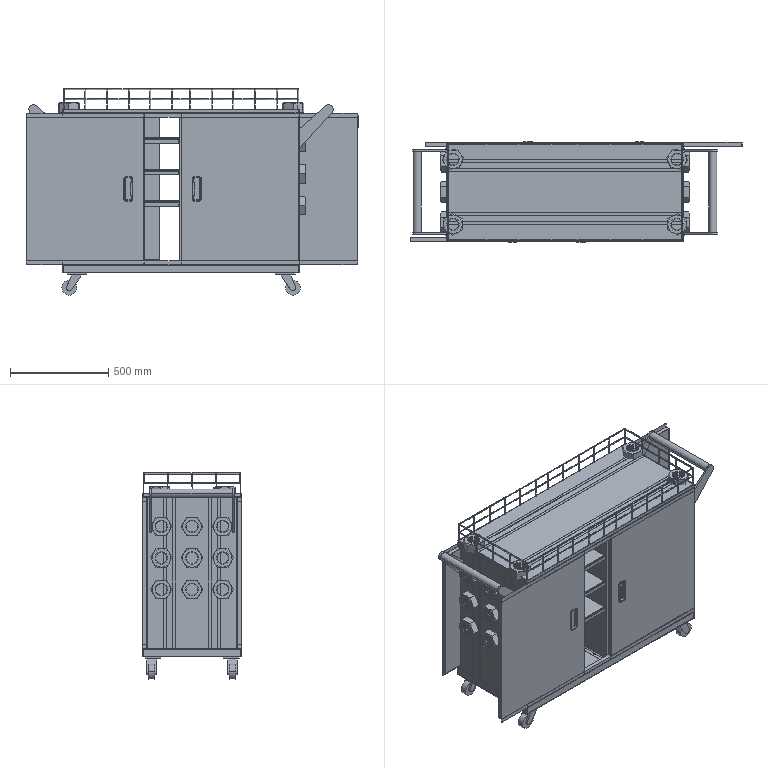Assembly | SolidWorks | mm | 67 component files | 67 solids | 4516 faces | box 1685.43 x 507.6 x 1046.33 mm | volume 19927785 mm3 | plane 1596 | cylinder 1476 | cone 1276 | torus 112 | spline 56 | commonest cylinder face diameters 57.505 x616 2 x198 5 x180 9 x112 8 x76 3.6 x74 20 x48 6 x28
Bill of materials:
BottomPlate | 1 | 304 | Plain flat rectangular plate of uniform thickness, with no visible holes or edge features.
ChassisFrame | 1 | Q235-A | Flat rectangular open lattice frame. It has a solid outer border, a long centre bar and a cross bar that form four large rectangular openings, and two small slot openings near each end. Shallow pads stick out from the underside near both ends.
Caster | 4 |  | Shape like a fixed caster: a rectangular top plate with four corner holes, a swept fork of two side plates angled down and back, and a solid cylindrical wheel held between the fork plates.
Handle | 4 |  | Rounded-rectangle plug or cap shape: a thin flange on one face with a slightly smaller rounded-rectangle body stepping out from it, and filleted corners.
InnerDoorPanel | 4 | 304 | Thin flat rectangular sheet panel with no visible holes. There may be very small returns at two opposite edges.
OuterDoorPanel | 4 | 304 | Thin rectangular sheet panel with slightly rounded corners and one rounded-rectangle slot near one vertical edge. Narrow bent flanges run along two opposite edges.
Fence | 1 | 304 | Rectangular perimeter railing of thin round rods: a continuous top rail and a mid rail around a rectangle, carried on evenly spaced vertical posts that extend below the mid rail.
GuideRailSchematic | 4 |  | Long straight prismatic bar with a square cross-section and plain flat ends.
Handle_2 | 2 |  | U-shaped handle-like part: a cylindrical cross bar between two flat side plates with rounded ends. The side plates are long and angled.
MiddleLowerConnectingPlate | 1 | 304 | Rectangular sheet panel with bent flanges along the top and bottom edges, each flange with three holes. The panel face has small holes near two corners along one edge.
MiddleUpperConnectingPlate | 1 | 304 | Rectangular sheet panel very similar to the previous flanged panel, with top and bottom flanges each holding three holes and small corner holes in the face. The flanges and edge return appear on the opposite side, so it may be a mirrored version.
Shelf | 6 | 304 | Shallow rectangular tray or shelf panel: a flat sheet with a short upturned lip along one long edge and a down-turned edge along the opposite long edge. That edge has three evenly spaced notches with rounded ends that are open at the bottom.
hexagon nuts grade c gb | 22 |  | Hexagonal nut with a central threaded through-bore and chamfered corners on both end faces.
TopPanelInnerPanel | 1 | 304 | Thin flat rectangular sheet plate with short upturned lips along two opposite long edges and small holes near both short ends.
TopPanelOuterPanel | 1 | 304 | Plain thin flat rectangular plate with no visible holes or formed features.
TopPanelStiffener | 2 | 304 | Long straight hat-section (omega) profile: two flat outer flanges in one plane with a recessed U-shaped central channel, all with rounded bends.
UpperLeftOuterSidePanel | 2 | 304 | Rectangular sheet panel with a narrow bent flange along one long edge. The flange has two round holes and appears shortened, with rounded corners at its ends.
UpperLeftOuterSidePanelInnerPanel | 2 | 304 | Rectangular sheet panel with a regular 3x3 grid of small round holes and short flanges bent along two opposite edges.
UpperLeftOuterSidePanelStiffener | 4 | 304 | Long straight hat-section profile with two coplanar outer flanges and an offset central web joined by rounded bends.
Mates:
1. coincident | CartChassis-1/BottomPlate-1 face at (-60.068, 34.625, 1223.05) dir (0, 0, 1) | UpperLeftSidePlate-1/UpperLeftOuterSidePanel-1 face at (539.132, 34.625, 1223.05) dir (0, 0, -1)
2. coincident | CartChassis-1/BottomPlate-1 face at (539.932, 34.625, 1222.25) dir (1, 0, 0) | UpperLeftSidePlate-1/UpperLeftOuterSidePanel-1 face at (539.932, 34.625, 1608.05) dir (1, 0, 0)
3. coincident | CartChassis-1/BottomPlate-1 face at (-60.068, 34.625, 1223.05) dir (0, 0, 1) | UpperLeftSidePlate-2/UpperLeftOuterSidePanel-1 face at (-659.268, 34.625, 1223.05) dir (0, 0, -1)
4. coincident | CartChassis-1/BottomPlate-1 face at (-660.068, 34.625, 1222.25) dir (-1, 0, 0) | UpperLeftSidePlate-2/UpperLeftOuterSidePanel-1 face at (-660.068, 34.625, 1608.05) dir (-1, 0, 0)
5. coincident | CartChassis-1/BottomPlate-1 face at (-60.068, 34.625, 1223.05) dir (0, 0, 1) | MiddleConnectingPlate-1/MiddleUpperConnectingPlate-1 face at (-70.068, 33.925, 1223.05) dir (0, 0, -1)
6. coincident | CartChassis-1/ChassisFrame-1 plane at (-59.368, 33.925, 1182.25) dir (0, 1, 0) | MiddleConnectingPlate-1/MiddleUpperConnectingPlate-1 plane at (-70.068, 33.925, 1608.05) dir (0, -1, 0)
7. coincident | UpperLeftSidePlate-2/UpperLeftOuterSidePanel-1 face at (-659.268, 34.625, 1993.05) dir (0, 0, 1) | TopPlate-1/TopPanelInnerPanel-2/TopPanelInnerPanel-1 face at (-659.068, -214.375, 1993.05) dir (0, 0, -1)
8. coincident | UpperLeftSidePlate-2/UpperLeftOuterSidePanel-1 face at (-660.068, 34.625, 1608.05) dir (-1, 0, 0) | TopPlate-1/TopPanelOuterPanel-1 face at (-660.068, 34.625, 2013.05) dir (-1, 0, 0)
9. coincident | CartChassis-1/BottomPlate-1 face at (-60.068, -215.375, 1222.25) dir (0, -1, 0) | TopPlate-1/TopPanelOuterPanel-1 face at (-60.068, -215.375, 2013.05) dir (0, -1, 0)
10. coincident | TopPlate-1/TopPanelInnerPanel-2/TopPanelInnerPanel-1 face at (-659.068, -214.375, 1993.05) dir (0, 0, -1) | DoorPlate-1/OuterDoorPanel-1 face at (238.386, 285.425, 1993.05) dir (0, 0, 1)
11. coincident | DoorPlate-1/OuterDoorPanel-1 face at (238.386, 285.425, 1993.05) dir (0, 1, 0) | DoorPlate-2/OuterDoorPanel-1 face at (-168.7, 285.425, 1223.05) dir (0, 1, 0)
12. coincident | DoorPlate-3/OuterDoorPanel-1 face at (-247.043, -216.175, 1993.05) dir (0, -1, 0) | DoorPlate-4/OuterDoorPanel-1 face at (-60.068, -216.175, 1223.05) dir (0, -1, 0)
13. coincident | DoorPlate-2/InnerDoorPanel-1 face at (-169.5, 266.125, 1973.05) dir (0, 0, 1) | DoorPlate-4/InnerDoorPanel-1 face at (-59.268, -196.875, 1973.05) dir (0, 0, 1)
14. coincident | UpperLeftSidePlate-1/UpperLeftOuterSidePanel-1 face at (539.932, 34.625, 1608.05) dir (1, 0, 0) | DoorPlate-4/OuterDoorPanel-1 face at (539.932, -215.375, 1223.05) dir (1, 0, 0)
15. coincident | CartChassis-1/BottomPlate-1 face at (-60.068, 34.625, 1223.05) dir (0, 0, 1) | GuideRailSchematic-1 face at (-660.068, 264.625, 1223.05) dir (0, 0, -1)
16. coincident | UpperLeftSidePlate-2/UpperLeftOuterSidePanel-1 face at (-660.068, 34.625, 1608.05) dir (-1, 0, 0) | GuideRailSchematic-1 face at (-660.068, 274.625, 1233.05) dir (-1, 0, 0)
17. coincident | DoorPlate-2/OuterDoorPanel-1 face at (-168.7, 284.625, 1223.05) dir (0, -1, 0) | GuideRailSchematic-1 face at (-660.068, 284.625, 1243.05) dir (0, 1, 0)
18. coincident | CartChassis-1/BottomPlate-1 face at (-60.068, 34.625, 1223.05) dir (0, 0, 1) | GuideRailSchematic-2 face at (-660.068, -215.375, 1223.05) dir (0, 0, -1)
19. coincident | UpperLeftSidePlate-2/UpperLeftOuterSidePanel-1 face at (-660.068, 34.625, 1608.05) dir (-1, 0, 0) | GuideRailSchematic-2 face at (-660.068, -205.375, 1233.05) dir (-1, 0, 0)
20. coincident | DoorPlate-3/OuterDoorPanel-1 face at (-247.043, -215.375, 1993.05) dir (0, 1, 0) | GuideRailSchematic-2 face at (-660.068, -215.375, 1243.05) dir (0, -1, 0)
21. coincident | DoorPlate-2/OuterDoorPanel-1 face at (-168.7, 284.625, 1223.05) dir (0, -1, 0) | GuideRailSchematic-4 face at (-660.068, 284.625, 1993.05) dir (0, 1, 0)
22. coincident | TopPlate-1/TopPanelInnerPanel-2/TopPanelInnerPanel-1 face at (-659.068, -214.375, 1993.05) dir (0, 0, -1) | GuideRailSchematic-4 face at (-660.068, 264.625, 1993.05) dir (0, 0, 1)
23. coincident | UpperLeftSidePlate-2/UpperLeftOuterSidePanel-1 face at (-660.068, 34.625, 1608.05) dir (-1, 0, 0) | GuideRailSchematic-4 face at (-660.068, 274.625, 1983.05) dir (-1, 0, 0)
24. coincident | DoorPlate-3/OuterDoorPanel-1 face at (-247.043, -215.375, 1993.05) dir (0, 1, 0) | GuideRailSchematic-3 face at (-660.068, -215.375, 1993.05) dir (0, -1, 0)
25. coincident | TopPlate-1/TopPanelInnerPanel-2/TopPanelInnerPanel-1 face at (-659.068, -214.375, 1993.05) dir (0, 0, -1) | GuideRailSchematic-3 face at (-660.068, -215.375, 1993.05) dir (0, 0, 1)
26. coincident | UpperLeftSidePlate-2/UpperLeftOuterSidePanel-1 face at (-660.068, 34.625, 1608.05) dir (-1, 0, 0) | GuideRailSchematic-3 face at (-660.068, -205.375, 1983.05) dir (-1, 0, 0)
27. coincident | UpperLeftSidePlate-1/UpperLeftOuterSidePanelInnerPanel-2/UpperLeftOuterSidePanelInnerPanel-1 face at (519.932, 34.625, 1608.05) dir (-1, 0, 0) | Shelf-1 face at (519.932, 23.375, 1858.25) dir (1, 0, 0)
28. coincident | Shelf-2 face at (234.932, 258.875, 1698.25) dir (0, 1, 0) | Shelf-3 face at (234.932, 258.875, 1538.25) dir (0, 1, 0)
29. coincident | Shelf-2 face at (-50.068, 23.375, 1698.25) dir (-1, 0, 0) | Shelf-3 face at (-50.068, 23.375, 1538.25) dir (-1, 0, 0)
30. concentric | UpperLeftSidePlate-1/UpperLeftOuterSidePanelInnerPanel-2/UpperLeftOuterSidePanelInnerPanel-1 face at (529.932, -120.875, 1844.55) dir (-1, 0, 0) r 4 | Shelf-1 face at (519.932, -120.875, 1844.55) dir (-1, 0, 0) r 4.5
31. concentric | UpperLeftSidePlate-1/UpperLeftOuterSidePanelInnerPanel-2/UpperLeftOuterSidePanelInnerPanel-1 face at (529.932, 34.625, 1844.55) dir (-1, 0, 0) r 4 | Shelf-1 face at (519.932, 34.625, 1844.55) dir (-1, 0, 0) r 4.5
32. coincident | Shelf-1 face at (234.932, 258.875, 1858.25) dir (0, 1, 0) | Shelf-2 face at (234.932, 258.875, 1698.25) dir (0, 1, 0)
33. coincident | UpperLeftSidePlate-1/UpperLeftOuterSidePanelInnerPanel-2/UpperLeftOuterSidePanelInnerPanel-1 face at (519.932, 34.625, 1608.05) dir (-1, 0, 0) | Shelf-2 face at (519.932, 23.375, 1698.25) dir (1, 0, 0)
34. concentric | UpperLeftSidePlate-1/UpperLeftOuterSidePanelInnerPanel-2/UpperLeftOuterSidePanelInnerPanel-1 face at (529.932, -120.875, 1684.55) dir (-1, 0, 0) r 4 | Shelf-2 face at (519.932, -120.875, 1684.55) dir (-1, 0, 0) r 4.5
35. concentric | UpperLeftSidePlate-1/UpperLeftOuterSidePanelInnerPanel-2/UpperLeftOuterSidePanelInnerPanel-1 face at (529.932, -120.875, 1524.55) dir (-1, 0, 0) r 4 | Shelf-3 face at (519.932, -120.875, 1524.55) dir (-1, 0, 0) r 4.5
36. coincident | Shelf-4 face at (-640.068, 23.375, 1858.25) dir (-1, 0, 0) | Shelf-5 face at (-640.068, 23.375, 1698.25) dir (-1, 0, 0)
37. coincident | Shelf-5 face at (-640.068, 23.375, 1698.25) dir (-1, 0, 0) | Shelf-6 face at (-640.068, 23.375, 1538.25) dir (-1, 0, 0)
38. coincident | Shelf-5 face at (-355.068, 258.875, 1698.25) dir (0, 1, 0) | Shelf-6 face at (-355.068, 258.875, 1538.25) dir (0, 1, 0)
39. coincident | Shelf-4 face at (-355.068, 258.875, 1858.25) dir (0, 1, 0) | Shelf-5 face at (-355.068, 258.875, 1698.25) dir (0, 1, 0)
40. coincident | MiddleConnectingPlate-1/MiddleUpperConnectingPlate-1 face at (-70.068, 33.925, 1608.05) dir (-1, 0, 0) | Shelf-6 face at (-70.068, 23.375, 1538.25) dir (1, 0, 0)
41. coincident | Shelf-2 face at (234.932, 258.875, 1698.25) dir (0, 1, 0) | Shelf-6 face at (-355.068, 258.875, 1538.25) dir (0, 1, 0)
42. coincident | Shelf-3 face at (234.932, 23.375, 1539.05) dir (0, 0, 1) | Shelf-6 face at (-355.068, 23.375, 1539.05) dir (0, 0, 1)
43. coincident | Shelf-2 face at (234.932, 23.375, 1699.05) dir (0, 0, 1) | Shelf-5 face at (-355.068, 23.375, 1699.05) dir (0, 0, 1)
44. coincident | Shelf-1 face at (234.932, 23.375, 1859.05) dir (0, 0, 1) | Shelf-4 face at (-355.068, 23.375, 1859.05) dir (0, 0, 1)
45. coincident | Caster-1 face at (424.132, 205.425, 1176.25) dir (0, 0, 1) | Caster-2 face at (424.132, -204.575, 1176.25) dir (0, 0, 1)
46. coincident | Caster-1 face at (424.132, 205.425, 1176.25) dir (-1, 0, 0) | Caster-2 face at (424.132, -204.575, 1176.25) dir (-1, 0, 0)
47. coincident | CartChassis-1/ChassisFrame-1 face at (519.132, 272.425, 1176.25) dir (1, 0, 0) | Caster-1 face at (519.132, 205.425, 1176.25) dir (1, 0, 0)
48. coincident | CartChassis-1/ChassisFrame-1 face at (-59.368, 33.925, 1176.25) dir (0, 0, -1) | Caster-2 face at (424.132, -204.575, 1176.25) dir (0, 0, 1)
49. coincident | CartChassis-1/ChassisFrame-1 face at (519.132, -204.575, 1176.25) dir (0, -1, 0) | Caster-2 face at (424.132, -204.575, 1171.25) dir (0, -1, 0)
50. coincident | CartChassis-1/ChassisFrame-1 face at (519.132, 272.425, 1176.25) dir (0, 1, 0) | Caster-1 face at (424.132, 272.425, 1171.25) dir (0, 1, 0)
51. coincident | Caster-3 face at (-542.868, -137.575, 1176.25) dir (0, 0, 1) | Caster-4 face at (-542.868, 272.425, 1176.25) dir (0, 0, 1)
52. coincident | Caster-3 face at (-637.868, -137.575, 1176.25) dir (-1, 0, 0) | Caster-4 face at (-637.868, 272.425, 1176.25) dir (-1, 0, 0)
53. coincident | CartChassis-1/ChassisFrame-1 face at (-59.368, 33.925, 1176.25) dir (0, 0, -1) | Caster-3 face at (-542.868, -137.575, 1176.25) dir (0, 0, 1)
54. coincident | CartChassis-1/ChassisFrame-1 face at (-637.868, 272.425, 1176.25) dir (-1, 0, 0) | Caster-3 face at (-637.868, -137.575, 1176.25) dir (-1, 0, 0)
55. coincident | CartChassis-1/ChassisFrame-1 face at (-637.868, -204.575, 1176.25) dir (0, -1, 0) | Caster-3 face at (-542.868, -204.575, 1171.25) dir (0, -1, 0)
56. coincident | CartChassis-1/ChassisFrame-1 face at (-637.868, 272.425, 1176.25) dir (0, 1, 0) | Caster-4 face at (-542.868, 272.425, 1171.25) dir (0, 1, 0)
57. coincident | TopPlate-1/TopPanelOuterPanel-1 face at (-60.068, 34.625, 2013.05) dir (0, 0, 1) | Fence-1 face at (-655.068, 157.125, 2013.05) dir (0, 0, -1)
58. symmetric | TopPlate-1/TopPanelOuterPanel-1 face at (-60.068, 284.625, 2013.05) dir (0, 1, 0) | TopPlate-1/TopPanelOuterPanel-1 face at (-60.068, -215.375, 2013.05) dir (0, -1, 0) | Fence-1 plane at (-60.068, 34.625, 2013.05) dir (0, 1, 0)
59. symmetric | TopPlate-1/TopPanelOuterPanel-1 face at (-660.068, 34.625, 2013.05) dir (-1, 0, 0) | TopPlate-1/TopPanelOuterPanel-1 face at (539.932, 34.625, 2013.05) dir (1, 0, 0) | Fence-1 plane at (-60.068, 34.625, 2013.05) dir (1, 0, 0)
60. symmetric | TopPlate-1/TopPanelOuterPanel-1 face at (-60.068, 284.625, 2013.05) dir (0, 1, 0) | TopPlate-1/TopPanelOuterPanel-1 face at (-60.068, -215.375, 2013.05) dir (0, -1, 0) | Handle_2-1 plane at (-660.068, 34.625, 1813.05) dir (0, 1, 0)
61. coincident | UpperLeftSidePlate-2/UpperLeftOuterSidePanel-1 face at (-660.068, 34.625, 1608.05) dir (-1, 0, 0) | Handle_2-1 face at (-660.068, 249.625, 1913.05) dir (1, 0, 0)
62. distance | Handle_2-1 edge at (-660.068, -170.375, 1913.05) dir (0, -1, 0) | TopPlate-1/TopPanelOuterPanel-1 face at (-60.068, 34.625, 2013.05) dir (0, 0, 1)
63. coincident | Handle_2-1 face at (-810.068, 249.625, 2013.05) dir (0, 1, 0) | Handle_2-2 face at (689.932, 249.625, 2013.05) dir (0, 1, 0)
64. coincident | UpperLeftSidePlate-1/UpperLeftOuterSidePanel-1 face at (539.932, 34.625, 1608.05) dir (1, 0, 0) | Handle_2-2 face at (539.932, -180.375, 1913.05) dir (-1, 0, 0)
65. distance | Handle_2-2 edge at (539.932, -180.375, 1913.05) dir (0, 1, 0) | TopPlate-1/TopPanelOuterPanel-1 face at (-60.068, 34.625, 2013.05) dir (0, 0, 1)
66. coincident | TopPlate-1/TopPanelOuterPanel-1 face at (-60.068, -215.375, 2013.05) dir (0, -1, 0) | DoorPlate-3/OuterDoorPanel-1 face at (-247.043, -215.375, 1993.05) dir (0, 1, 0)
67. coincident | TopPlate-1/TopPanelOuterPanel-1 face at (-60.068, 284.625, 2013.05) dir (0, 1, 0) | DoorPlate-1/OuterDoorPanel-1 face at (238.386, 284.625, 1993.05) dir (0, -1, 0)
68. coincident | CartChassis-1/BottomPlate-1 plane at (-60.068, 34.625, 1222.25) dir (0, -1, 0) | UpperLeftSidePlate-1 plane at (539.132, 34.625, 1608.05) dir (0, 1, 0)
69. coincident | CartChassis-1/BottomPlate-1 plane at (-60.068, 34.625, 1222.25) dir (0, -1, 0) | UpperLeftSidePlate-2 plane at (-659.268, 34.625, 1608.05) dir (0, -1, 0)
70. symmetric | CartChassis-1/BottomPlate-1 plane at (-60.068, 34.625, 1222.25) dir (1, 0, 0) | MiddleConnectingPlate-1/MiddleUpperConnectingPlate-1 face at (-70.068, 33.925, 1608.05) dir (-1, 0, 0) | MiddleConnectingPlate-1/MiddleLowerConnectingPlate-1 face at (-50.068, 33.925, 1608.05) dir (1, 0, 0)
71. coincident | TopPlate-1/TopPanelInnerPanel-2/TopPanelInnerPanel-1 face at (-659.068, -214.375, 1993.05) dir (0, 0, -1) | DoorPlate-2/OuterDoorPanel-1 face at (-168.7, 284.625, 1993.05) dir (0, 0, 1)
72. coincident | DoorPlate-1/InnerDoorPanel-1 face at (239.186, 266.125, 1970.05) dir (0, 0, 1) | DoorPlate-3/InnerDoorPanel-1 face at (-247.843, -196.875, 1970.05) dir (0, 0, 1)
73. coincident | ChassisFrame-1 face at (-544.114, -212.243, 1220) dir (0, -1, 0) | BottomPlate-1 face at (53.686, -212.243, 1220) dir (0, 1, 0)
74. coincident | ChassisFrame-1 face at (652.886, -212.243, 1220) dir (1, 0, 0) | BottomPlate-1 face at (652.886, 36.957, 1220) dir (-1, 0, 0)
75. coincident | ChassisFrame-1 face at (54.386, 36.257, 1220) dir (0, 0, 1) | BottomPlate-1 face at (53.686, 36.957, 1220) dir (0, 0, -1)
76. coincident | OuterDoorPanel-1 face at (49.311, -288.312, 1030) dir (-1, 0, 0) | InnerDoorPanel-1 face at (49.311, 461.688, 1029.2) dir (1, 0, 0)
77. coincident | OuterDoorPanel-1 face at (49.311, -288.312, 1029.2) dir (0, 0, -1) | InnerDoorPanel-1 face at (30.011, -265.312, 1029.2) dir (0, 0, 1)
78. coincident | OuterDoorPanel-1 face at (29.311, 461.688, 430) dir (0, 1, 0) | InnerDoorPanel-1 face at (30.811, 461.688, 1029.2) dir (0, 1, 0)
79. coincident | OuterDoorPanel-1 face at (29.31, 46.688, 970) dir (0, 0, -1) | Handle-1 face at (50.111, 146.688, 970) dir (0, 0, 1)
80. coincident | OuterDoorPanel-1 face at (29.31, 156.688, 940) dir (0, -1, 0) | Handle-1 face at (50.111, 156.688, 960) dir (0, 1, 0)
81. coincident | OuterDoorPanel-1 face at (50.111, -288.312, 1030) dir (1, 0, 0) | Handle-1 face at (50.111, 146.688, 960) dir (-1, 0, 0)
82. width | MiddleLowerConnectingPlate-1 face at (0, -19.2, -226.2) dir (0, 0, 1) | MiddleLowerConnectingPlate-1 face at (0, -19.2, 226.2) dir (0, 0, -1) | MiddleUpperConnectingPlate-1 face at (0, 0, -228.5) dir (0, 0, -1) | MiddleUpperConnectingPlate-1 face at (0, 0, 228.5) dir (0, 0, 1)
83. coincident | MiddleUpperConnectingPlate-1 face at (-385, 0, 0) dir (-1, 0, 0) | MiddleLowerConnectingPlate-1 face at (-385, -19.2, 0) dir (-1, 0, 0)
84. distance | MiddleLowerConnectingPlate-1 face at (0, -20, 0) dir (0, -1, 0) | MiddleUpperConnectingPlate-1 face at (0, 0, 0) dir (0, 1, 0)
85. coincident | TopPanelOuterPanel-1 face at (0, -0.8, 0) dir (0, -1, 0) | TopPanelStiffener-1 face at (-598, -0.8, 165) dir (0, 1, 0)
86. width | TopPanelOuterPanel-1 face at (-599.2, 0, 0) dir (1, 0, 0) | TopPanelOuterPanel-1 face at (599.2, 0, 0) dir (-1, 0, 0) | TopPanelStiffener-1 face at (-598, -17.4, 149.2) dir (-1, 0, 0) | TopPanelStiffener-1 face at (598, -17.4, 120.8) dir (1, 0, 0)
87. distance | TopPanelStiffener-1 face at (-598, -1.6, 150) dir (0, 0, 1) | TopPanelOuterPanel-1 face at (0, 0, 250) dir (0, 0, 1)
88. coincident | TopPanelOuterPanel-1 face at (0, -0.8, 0) dir (0, -1, 0) | TopPanelStiffener-2 face at (-598, -0.8, -105) dir (0, 1, 0)
89. width | TopPanelOuterPanel-1 face at (599.2, 0, 0) dir (-1, 0, 0) | TopPanelOuterPanel-1 face at (-599.2, 0, 0) dir (1, 0, 0) | TopPanelStiffener-2 face at (-598, -18.4, -148.2) dir (-1, 0, 0) | TopPanelStiffener-2 face at (598, -0.8, -151) dir (1, 0, 0)
90. parallel | TopPanelOuterPanel-1 face at (0, -0.8, 0) dir (0, -1, 0) | TopPanelInnerPanel-2/TopPanelInnerPanel-1 face at (-599, -19.2, 249) dir (0, 1, 0)
91. width | TopPanelOuterPanel-1 face at (0, 0, -250) dir (0, 0, -1) | TopPanelOuterPanel-1 face at (0, 0, 250) dir (0, 0, 1) | TopPanelInnerPanel-2/TopPanelInnerPanel-1 face at (-599, -1.5, 249) dir (0, 0, 1) | TopPanelInnerPanel-2/TopPanelInnerPanel-1 face at (-599, -1.5, -249) dir (0, 0, -1)
92. width | TopPanelOuterPanel-1 face at (600, 0, 0) dir (1, 0, 0) | TopPanelOuterPanel-1 face at (-600, 0, 0) dir (-1, 0, 0) | TopPanelInnerPanel-2/TopPanelInnerPanel-1 face at (-599, -18.2, 248.2) dir (-1, 0, 0) | TopPanelInnerPanel-2/TopPanelInnerPanel-1 face at (599, -18.2, -248.2) dir (1, 0, 0)
93. distance | TopPanelOuterPanel-1 face at (0, 0, -250) dir (0, 0, -1) | TopPanelStiffener-2 face at (-598, -1.6, -150) dir (0, 0, -1)
94. coincident | TopPanelStiffener-1 face at (-598, -19.2, 150) dir (0, -1, 0) | TopPanelInnerPanel-2/TopPanelInnerPanel-1 face at (-599, -19.2, 249) dir (0, 1, 0)
95. coincident | TopPanelInnerPanel-1 face at (-249, 599, 0.8) dir (0, 0, 1) | hexagon nuts grade c gb-5 face at (-192.424, -521.5, 0.8) dir (0, 0, -1)
96. coincident | TopPanelInnerPanel-1 face at (-249, 599, 0.8) dir (0, 0, 1) | hexagon nuts grade c gb-7 face at (157.862, -623.382, 0.8) dir (0, 0, -1)
97. concentric | TopPanelInnerPanel-1 face at (-165, -569, 10) dir (0, 0, -1) r 4 | hexagon nuts grade c gb-5 edge at (-165, -569, 0.8) dir (0, 0, 1) r 3.324
98. concentric | TopPanelInnerPanel-1 face at (165, -569, 10) dir (0, 0, -1) r 4 | hexagon nuts grade c gb-7 face at (165, -569, 53.2) dir (0, 0, -1) r 28.753
99. coincident | UpperLeftOuterSidePanel-1 face at (0, 0, 0) dir (0, 1, 0) | UpperLeftOuterSidePanelStiffener-1 face at (-84.5, 0, 383) dir (0, -1, 0)
100. width | UpperLeftOuterSidePanel-1 face at (0, 0, -384.2) dir (0, 0, 1) | UpperLeftOuterSidePanel-1 face at (0, 0, 384.2) dir (0, 0, -1) | UpperLeftOuterSidePanelStiffener-1 face at (-102, 16.9, 383) dir (0, 0, 1) | UpperLeftOuterSidePanelStiffener-1 face at (-98.5, 0, -383) dir (0, 0, -1)
101. distance | UpperLeftOuterSidePanelStiffener-1 face at (-129.5, 1.5, 383) dir (-1, 0, 0) | UpperLeftOuterSidePanel-1 face at (-229.5, 0, 0) dir (-1, 0, 0)
102. coincident | UpperLeftOuterSidePanel-1 face at (0, 0, 0) dir (0, 1, 0) | UpperLeftOuterSidePanelStiffener-2 face at (84.5, 0, 383) dir (0, -1, 0)
103. width | UpperLeftOuterSidePanel-1 face at (0, 0, -384.2) dir (0, 0, 1) | UpperLeftOuterSidePanel-1 face at (0, 0, 384.2) dir (0, 0, -1) | UpperLeftOuterSidePanelStiffener-2 face at (102, 16.9, -383) dir (0, 0, -1) | UpperLeftOuterSidePanelStiffener-2 face at (99.5, 2.5, 383) dir (0, 0, 1)
104. width | UpperLeftOuterSidePanel-1 face at (-229.5, 0, 0) dir (-1, 0, 0) | UpperLeftOuterSidePanel-1 face at (229.5, 0, 0) dir (1, 0, 0) | UpperLeftOuterSidePanelInnerPanel-2/UpperLeftOuterSidePanelInnerPanel-1 face at (228, 19.2, 0) dir (1, 0, 0) | UpperLeftOuterSidePanelInnerPanel-2/UpperLeftOuterSidePanelInnerPanel-1 face at (-228, 19.2, 0) dir (-1, 0, 0)
105. width | UpperLeftOuterSidePanel-1 face at (0, 0, 385) dir (0, 0, 1) | UpperLeftOuterSidePanel-1 face at (0, 0, -385) dir (0, 0, -1) | UpperLeftOuterSidePanelInnerPanel-2/UpperLeftOuterSidePanelInnerPanel-1 face at (-228, 18.4, -383.5) dir (0, 0, -1) | UpperLeftOuterSidePanelInnerPanel-2/UpperLeftOuterSidePanelInnerPanel-1 face at (-228, 18.4, 383.5) dir (0, 0, 1)
106. distance | UpperLeftOuterSidePanel-1 face at (229.5, 0, 0) dir (1, 0, 0) | UpperLeftOuterSidePanelStiffener-2 face at (129.5, 1.5, 383) dir (1, 0, 0)
107. coincident | UpperLeftOuterSidePanelStiffener-1 face at (-129.5, 18.4, 383) dir (0, 1, 0) | UpperLeftOuterSidePanelInnerPanel-2/UpperLeftOuterSidePanelInnerPanel-1 face at (0, 18.4, 0) dir (0, -1, 0)
108. coincident | UpperLeftOuterSidePanelInnerPanel-1 face at (0, -0.8, 0) dir (0, -1, 0) | hexagon nuts grade c gb-16 face at (182.924, -0.8, -36) dir (0, 1, 0)
109. coincident | UpperLeftOuterSidePanelInnerPanel-1 face at (0, -0.8, 0) dir (0, -1, 0) | hexagon nuts grade c gb-19 face at (182.924, -0.8, 124) dir (0, 1, 0)
110. coincident | UpperLeftOuterSidePanelInnerPanel-1 face at (0, -0.8, 0) dir (0, -1, 0) | hexagon nuts grade c gb-22 face at (182.924, -0.8, 284) dir (0, 1, 0)
111. concentric | UpperLeftOuterSidePanelInnerPanel-1 face at (155.5, -10, -83.5) dir (0, 1, 0) r 4 | hexagon nuts grade c gb-16 edge at (155.5, -8.7, -83.5) dir (0, 1, 0) r 3.324
112. concentric | UpperLeftOuterSidePanelInnerPanel-1 face at (155.5, -10, 76.5) dir (0, 1, 0) r 4 | hexagon nuts grade c gb-19 face at (155.5, -53.2, 76.5) dir (0, 1, 0) r 28.753
113. concentric | UpperLeftOuterSidePanelInnerPanel-1 edge at (155.5, -0.8, 236.5) dir (0, -1, 0) r 4 | hexagon nuts grade c gb-22 edge at (155.5, -8.7, 236.5) dir (0, 1, 0) r 3.324